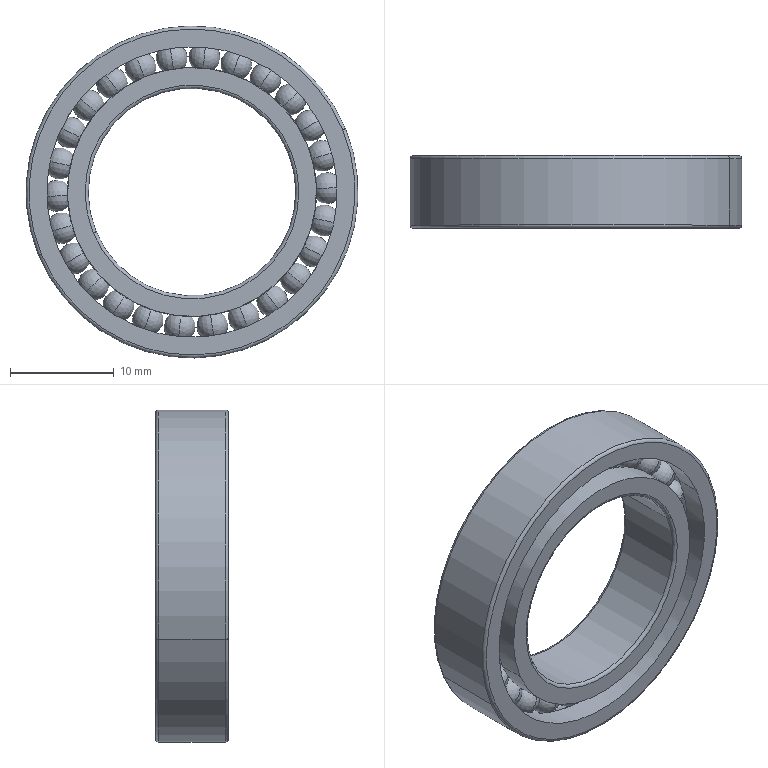Component | SolidWorks | DialAxis-1_deep groove ball bearings gb-2 | 1 solid | 157 faces | volume 2526 mm3 | torus 89 | sphere 52 | cylinder 12 | plane 4 | commonest cylinder face diameters 28 x4 24 x4 32 x2 20 x2